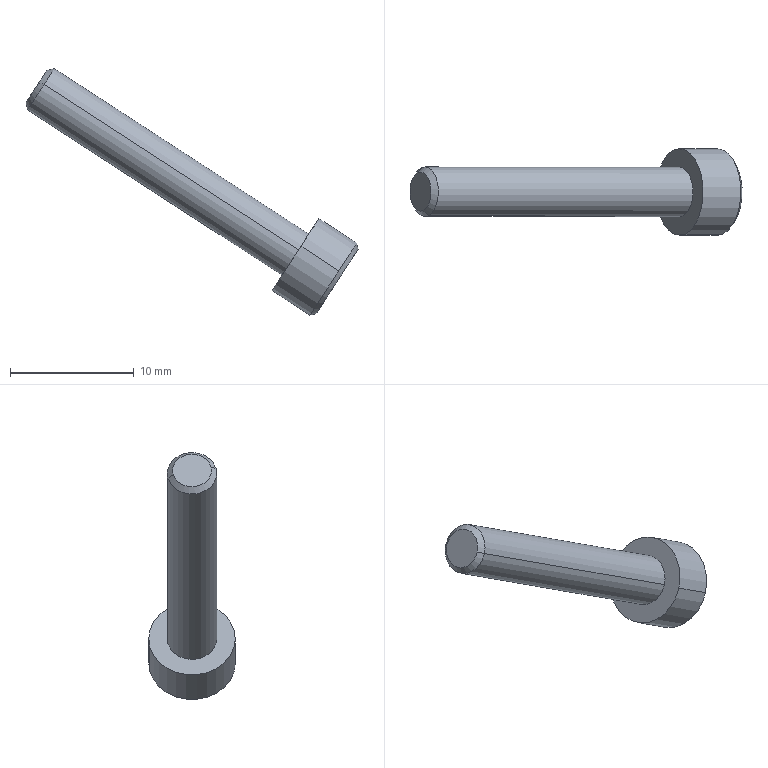Component | SolidWorks | ScrewTAC21-M4-L25(YIHEDA)-1 | 1 solid | 25 faces | box 26.89 x 7 x 19.98 mm | volume 448 mm3 | plane 15 | cone 6 | cylinder 4 | commonest cylinder face diameters 7 x2 4 x2
STEP:
#1=CARTESIAN_POINT('',(3.54,-0.8802,10.973));
#2=VERTEX_POINT('',#1);
#3=CARTESIAN_POINT('',(3.556,-1.,10.997));
#4=VERTEX_POINT('',#3);
#5=CARTESIAN_POINT('',(3.548,-0.9403,10.985));
#6=DIRECTION('',(-0.8387,0.,0.5446));
#7=DIRECTION('',(-0.1266,0.9726,-0.195));
#8=AXIS2_PLACEMENT_3D('',#5,#6,#7);
#9=CIRCLE('',#8,0.06183);
#10=EDGE_CURVE('',#2,#4,#9,.T.);
#11=ORIENTED_EDGE('',*,*,#10,.F.);
#12=CARTESIAN_POINT('',(3.552,-0.8637,10.961));
#13=VERTEX_POINT('',#12);
#14=CARTESIAN_POINT('',(3.552,-0.8637,10.961));
#15=DIRECTION('',(0.5035,0.6877,-0.523));
#16=VECTOR('',#15,39.37);
#17=LINE('',#14,#16);
#18=EDGE_CURVE('',#2,#13,#17,.T.);
#19=ORIENTED_EDGE('',*,*,#18,.T.);
#20=CARTESIAN_POINT('',(3.572,-1.017,10.991));
#21=VERTEX_POINT('',#20);
#22=CARTESIAN_POINT('',(3.562,-0.9403,10.976));
#23=DIRECTION('',(-0.8387,0.,0.5446));
#24=DIRECTION('',(-0.1266,0.9726,-0.195));
#25=AXIS2_PLACEMENT_3D('',#22,#23,#24);
#26=CIRCLE('',#25,0.07874);
#27=EDGE_CURVE('',#13,#21,#26,.T.);
#28=ORIENTED_EDGE('',*,*,#27,.T.);
#29=CARTESIAN_POINT('',(3.572,-1.017,10.991));
#30=DIRECTION('',(0.6826,-0.6877,-0.2473));
#31=VECTOR('',#30,39.37);
#32=LINE('',#29,#31);
#33=EDGE_CURVE('',#4,#21,#32,.T.);
#34=ORIENTED_EDGE('',*,*,#33,.F.);
#35=EDGE_LOOP('',(#11,#19,#28,#34));
#36=FACE_OUTER_BOUND('',#35,.T.);
#37=CARTESIAN_POINT('',(3.562,-0.9403,10.976));
#38=DIRECTION('',(0.8387,-0.,-0.5446));
#39=DIRECTION('',(0.1266,-0.9726,0.195));
#40=AXIS2_PLACEMENT_3D('',#37,#38,#39);
#41=CONICAL_SURFACE('',#40,0.07874,0.7854);
#42=ADVANCED_FACE('',(#36),#41,.T.);
#43=CARTESIAN_POINT('',(4.49,-0.8197,10.339));
#44=VERTEX_POINT('',#43);
#45=CARTESIAN_POINT('',(4.521,-1.061,10.388));
#46=VERTEX_POINT('',#45);
#47=CARTESIAN_POINT('',(4.506,-0.9403,10.363));
#48=DIRECTION('',(-0.8387,0.,0.5446));
#49=DIRECTION('',(-0.1266,0.9726,-0.195));
#50=AXIS2_PLACEMENT_3D('',#47,#48,#49);
#51=CIRCLE('',#50,0.124);
#52=EDGE_CURVE('',#44,#46,#51,.T.);
#53=ORIENTED_EDGE('',*,*,#52,.T.);
#54=CARTESIAN_POINT('',(4.512,-1.074,10.398));
#55=VERTEX_POINT('',#54);
#56=CARTESIAN_POINT('',(4.521,-1.061,10.388));
#57=DIRECTION('',(-0.5035,-0.6877,0.523));
#58=VECTOR('',#57,39.37);
#59=LINE('',#56,#58);
#60=EDGE_CURVE('',#46,#55,#59,.T.);
#61=ORIENTED_EDGE('',*,*,#60,.T.);
#62=CARTESIAN_POINT('',(4.477,-0.8063,10.344));
#63=VERTEX_POINT('',#62);
#64=CARTESIAN_POINT('',(4.494,-0.9403,10.371));
#65=DIRECTION('',(-0.8387,0.,0.5446));
#66=DIRECTION('',(-0.1266,0.9726,-0.195));
#67=AXIS2_PLACEMENT_3D('',#64,#65,#66);
#68=CIRCLE('',#67,0.1378);
#69=EDGE_CURVE('',#63,#55,#68,.T.);
#70=ORIENTED_EDGE('',*,*,#69,.F.);
#71=CARTESIAN_POINT('',(4.49,-0.8197,10.339));
#72=DIRECTION('',(-0.6826,0.6877,0.2473));
#73=VECTOR('',#72,39.37);
#74=LINE('',#71,#73);
#75=EDGE_CURVE('',#44,#63,#74,.T.);
#76=ORIENTED_EDGE('',*,*,#75,.F.);
#77=EDGE_LOOP('',(#53,#61,#70,#76));
#78=FACE_OUTER_BOUND('',#77,.T.);
#79=CARTESIAN_POINT('',(4.506,-0.9403,10.363));
#80=DIRECTION('',(-0.8387,0.,0.5446));
#81=DIRECTION('',(-0.1266,0.9726,-0.195));
#82=AXIS2_PLACEMENT_3D('',#79,#80,#81);
#83=CONICAL_SURFACE('',#82,0.124,0.7854);
#84=ADVANCED_FACE('',(#78),#83,.T.);
#85=CARTESIAN_POINT('',(4.391,-1.074,10.476));
#86=VERTEX_POINT('',#85);
#87=CARTESIAN_POINT('',(4.356,-0.8063,10.422));
#88=VERTEX_POINT('',#87);
#89=CARTESIAN_POINT('',(4.374,-0.9403,10.449));
#90=DIRECTION('',(-0.8387,0.,0.5446));
#91=DIRECTION('',(-0.1266,0.9726,-0.195));
#92=AXIS2_PLACEMENT_3D('',#89,#90,#91);
#93=CIRCLE('',#92,0.1378);
#94=EDGE_CURVE('',#86,#88,#93,.T.);
#95=ORIENTED_EDGE('',*,*,#94,.F.);
#96=CARTESIAN_POINT('',(4.391,-1.074,10.476));
#97=DIRECTION('',(0.8387,-0.,-0.5446));
#98=VECTOR('',#97,39.37);
#99=LINE('',#96,#98);
#100=EDGE_CURVE('',#86,#55,#99,.T.);
#101=ORIENTED_EDGE('',*,*,#100,.T.);
#102=CARTESIAN_POINT('',(4.494,-0.9403,10.371));
#103=DIRECTION('',(-0.8387,0.,0.5446));
#104=DIRECTION('',(-0.1266,0.9726,-0.195));
#105=AXIS2_PLACEMENT_3D('',#102,#103,#104);
#106=CIRCLE('',#105,0.1378);
#107=EDGE_CURVE('',#55,#63,#106,.T.);
#108=ORIENTED_EDGE('',*,*,#107,.T.);
#109=CARTESIAN_POINT('',(4.356,-0.8063,10.422));
#110=DIRECTION('',(0.8387,-0.,-0.5446));
#111=VECTOR('',#110,39.37);
#112=LINE('',#109,#111);
#113=EDGE_CURVE('',#88,#63,#112,.T.);
#114=ORIENTED_EDGE('',*,*,#113,.F.);
#115=EDGE_LOOP('',(#95,#101,#108,#114));
#116=FACE_OUTER_BOUND('',#115,.T.);
#117=CARTESIAN_POINT('',(4.374,-0.9403,10.449));
#118=DIRECTION('',(0.8387,-0.,-0.5446));
#119=DIRECTION('',(-0.1266,0.9726,-0.195));
#120=AXIS2_PLACEMENT_3D('',#117,#118,#119);
#121=CYLINDRICAL_SURFACE('',#120,0.1378);
#122=ADVANCED_FACE('',(#116),#121,.T.);
#123=CARTESIAN_POINT('',(4.411,-0.9403,10.425));
#124=VERTEX_POINT('',#123);
#125=CARTESIAN_POINT('',(4.471,-0.9266,10.454));
#126=VERTEX_POINT('',#125);
#127=CARTESIAN_POINT('',(4.471,-0.9266,10.454));
#128=DIRECTION('',(0.8781,0.2013,0.4341));
#129=VECTOR('',#128,39.37);
#130=LINE('',#127,#129);
#131=EDGE_CURVE('',#124,#126,#130,.T.);
#132=ORIENTED_EDGE('',*,*,#131,.F.);
#133=CARTESIAN_POINT('',(4.408,-0.954,10.358));
#134=VERTEX_POINT('',#133);
#135=CARTESIAN_POINT('',(4.408,-0.954,10.358));
#136=DIRECTION('',(-0.03941,-0.2013,-0.9787));
#137=VECTOR('',#136,39.37);
#138=LINE('',#135,#137);
#139=EDGE_CURVE('',#124,#134,#138,.T.);
#140=ORIENTED_EDGE('',*,*,#139,.T.);
#141=CARTESIAN_POINT('',(4.409,-0.9235,10.359));
#142=VERTEX_POINT('',#141);
#143=CARTESIAN_POINT('',(4.44,-0.9403,10.406));
#144=DIRECTION('',(-0.8387,0.,0.5446));
#145=DIRECTION('',(0.1266,-0.9726,0.195));
#146=AXIS2_PLACEMENT_3D('',#143,#144,#145);
#147=CIRCLE('',#146,0.05906);
#148=EDGE_CURVE('',#142,#134,#147,.T.);
#149=ORIENTED_EDGE('',*,*,#148,.F.);
#150=CARTESIAN_POINT('',(4.432,-0.8829,10.395));
#151=VERTEX_POINT('',#150);
#152=CARTESIAN_POINT('',(4.44,-0.9403,10.406));
#153=DIRECTION('',(-0.8387,0.,0.5446));
#154=DIRECTION('',(0.1266,-0.9726,0.195));
#155=AXIS2_PLACEMENT_3D('',#152,#153,#154);
#156=CIRCLE('',#155,0.05906);
#157=EDGE_CURVE('',#151,#142,#156,.T.);
#158=ORIENTED_EDGE('',*,*,#157,.F.);
#159=CARTESIAN_POINT('',(4.463,-0.8997,10.442));
#160=VERTEX_POINT('',#159);
#161=CARTESIAN_POINT('',(4.44,-0.9403,10.406));
#162=DIRECTION('',(-0.8387,0.,0.5446));
#163=DIRECTION('',(0.1266,-0.9726,0.195));
#164=AXIS2_PLACEMENT_3D('',#161,#162,#163);
#165=CIRCLE('',#164,0.05906);
#166=EDGE_CURVE('',#160,#151,#165,.T.);
#167=ORIENTED_EDGE('',*,*,#166,.F.);
#168=CARTESIAN_POINT('',(4.44,-0.9403,10.406));
#169=DIRECTION('',(-0.8387,0.,0.5446));
#170=DIRECTION('',(0.1266,-0.9726,0.195));
#171=AXIS2_PLACEMENT_3D('',#168,#169,#170);
#172=CIRCLE('',#171,0.05906);
#173=EDGE_CURVE('',#126,#160,#172,.T.);
#174=ORIENTED_EDGE('',*,*,#173,.F.);
#175=EDGE_LOOP('',(#132,#140,#149,#158,#167,#174));
#176=FACE_OUTER_BOUND('',#175,.T.);
#177=CARTESIAN_POINT('',(4.44,-0.9403,10.406));
#178=DIRECTION('',(0.8387,-0.,-0.5446));
#179=DIRECTION('',(0.5297,0.2325,0.8157));
#180=AXIS2_PLACEMENT_3D('',#177,#178,#179);
#181=CONICAL_SURFACE('',#180,0.05906,1.047);
#182=ADVANCED_FACE('',(#176),#181,.F.);
#183=CARTESIAN_POINT('',(3.562,-0.9403,10.976));
#184=DIRECTION('',(-0.8387,0.,0.5446));
#185=DIRECTION('',(-0.1266,0.9726,-0.195));
#186=AXIS2_PLACEMENT_3D('',#183,#184,#185);
#187=CIRCLE('',#186,0.07874);
#188=EDGE_CURVE('',#21,#13,#187,.T.);
#189=ORIENTED_EDGE('',*,*,#188,.F.);
#190=CARTESIAN_POINT('',(4.384,-1.017,10.465));
#191=VERTEX_POINT('',#190);
#192=CARTESIAN_POINT('',(3.558,-1.017,11.001));
#193=DIRECTION('',(0.8387,-0.,-0.5446));
#194=VECTOR('',#193,39.37);
#195=LINE('',#192,#194);
#196=EDGE_CURVE('',#21,#191,#195,.T.);
#197=ORIENTED_EDGE('',*,*,#196,.T.);
#198=CARTESIAN_POINT('',(4.364,-0.8637,10.434));
#199=VERTEX_POINT('',#198);
#200=CARTESIAN_POINT('',(4.374,-0.9403,10.449));
#201=DIRECTION('',(-0.8387,0.,0.5446));
#202=DIRECTION('',(-0.1266,0.9726,-0.195));
#203=AXIS2_PLACEMENT_3D('',#200,#201,#202);
#204=CIRCLE('',#203,0.07874);
#205=EDGE_CURVE('',#191,#199,#204,.T.);
#206=ORIENTED_EDGE('',*,*,#205,.T.);
#207=CARTESIAN_POINT('',(3.538,-0.8637,10.97));
#208=DIRECTION('',(0.8387,-0.,-0.5446));
#209=VECTOR('',#208,39.37);
#210=LINE('',#207,#209);
#211=EDGE_CURVE('',#13,#199,#210,.T.);
#212=ORIENTED_EDGE('',*,*,#211,.F.);
#213=EDGE_LOOP('',(#189,#197,#206,#212));
#214=FACE_OUTER_BOUND('',#213,.T.);
#215=CARTESIAN_POINT('',(3.548,-0.9403,10.985));
#216=DIRECTION('',(0.8387,-0.,-0.5446));
#217=DIRECTION('',(-0.1266,0.9726,-0.195));
#218=AXIS2_PLACEMENT_3D('',#215,#216,#217);
#219=CYLINDRICAL_SURFACE('',#218,0.07874);
#220=ADVANCED_FACE('',(#214),#219,.T.);
#221=CARTESIAN_POINT('',(4.476,-0.9245,10.462));
#222=VERTEX_POINT('',#221);
#223=CARTESIAN_POINT('',(4.471,-0.9571,10.454));
#224=VERTEX_POINT('',#223);
#225=CARTESIAN_POINT('',(4.476,-0.9245,10.462));
#226=DIRECTION('',(-0.1552,-0.9585,-0.239));
#227=VECTOR('',#226,39.37);
#228=LINE('',#225,#227);
#229=EDGE_CURVE('',#222,#224,#228,.T.);
#230=ORIENTED_EDGE('',*,*,#229,.T.);
#231=CARTESIAN_POINT('',(4.44,-0.9403,10.406));
#232=DIRECTION('',(-0.8387,0.,0.5446));
#233=DIRECTION('',(0.1266,-0.9726,0.195));
#234=AXIS2_PLACEMENT_3D('',#231,#232,#233);
#235=CIRCLE('',#234,0.05906);
#236=EDGE_CURVE('',#224,#126,#235,.T.);
#237=ORIENTED_EDGE('',*,*,#236,.T.);
#238=ORIENTED_EDGE('',*,*,#173,.T.);
#239=CARTESIAN_POINT('',(4.45,-0.875,10.423));
#240=DIRECTION('',(0.3745,-0.7261,0.5767));
#241=VECTOR('',#240,39.37);
#242=LINE('',#239,#241);
#243=EDGE_CURVE('',#160,#222,#242,.T.);
#244=ORIENTED_EDGE('',*,*,#243,.T.);
#245=EDGE_LOOP('',(#230,#237,#238,#244));
#246=FACE_OUTER_BOUND('',#245,.T.);
#247=CARTESIAN_POINT('',(4.44,-0.9403,10.406));
#248=DIRECTION('',(0.8387,-0.,-0.5446));
#249=DIRECTION('',(0.1266,-0.9726,0.195));
#250=AXIS2_PLACEMENT_3D('',#247,#248,#249);
#251=PLANE('',#250);
#252=ADVANCED_FACE('',(#246),#251,.T.);
#253=ORIENTED_EDGE('',*,*,#196,.F.);
#254=ORIENTED_EDGE('',*,*,#27,.F.);
#255=ORIENTED_EDGE('',*,*,#211,.T.);
#256=CARTESIAN_POINT('',(4.374,-0.9403,10.449));
#257=DIRECTION('',(-0.8387,0.,0.5446));
#258=DIRECTION('',(-0.1266,0.9726,-0.195));
#259=AXIS2_PLACEMENT_3D('',#256,#257,#258);
#260=CIRCLE('',#259,0.07874);
#261=EDGE_CURVE('',#199,#191,#260,.T.);
#262=ORIENTED_EDGE('',*,*,#261,.T.);
#263=EDGE_LOOP('',(#253,#254,#255,#262));
#264=FACE_OUTER_BOUND('',#263,.T.);
#265=CARTESIAN_POINT('',(3.548,-0.9403,10.985));
#266=DIRECTION('',(0.8387,-0.,-0.5446));
#267=DIRECTION('',(-0.1266,0.9726,-0.195));
#268=AXIS2_PLACEMENT_3D('',#265,#266,#267);
#269=CYLINDRICAL_SURFACE('',#268,0.07874);
#270=ADVANCED_FACE('',(#264),#269,.T.);
#271=ORIENTED_EDGE('',*,*,#139,.F.);
#272=ORIENTED_EDGE('',*,*,#131,.T.);
#273=ORIENTED_EDGE('',*,*,#236,.F.);
#274=CARTESIAN_POINT('',(4.447,-0.9978,10.418));
#275=VERTEX_POINT('',#274);
#276=CARTESIAN_POINT('',(4.44,-0.9403,10.406));
#277=DIRECTION('',(-0.8387,0.,0.5446));
#278=DIRECTION('',(0.1266,-0.9726,0.195));
#279=AXIS2_PLACEMENT_3D('',#276,#277,#278);
#280=CIRCLE('',#279,0.05906);
#281=EDGE_CURVE('',#275,#224,#280,.T.);
#282=ORIENTED_EDGE('',*,*,#281,.F.);
#283=CARTESIAN_POINT('',(4.416,-0.9809,10.37));
#284=VERTEX_POINT('',#283);
#285=CARTESIAN_POINT('',(4.44,-0.9403,10.406));
#286=DIRECTION('',(-0.8387,0.,0.5446));
#287=DIRECTION('',(0.1266,-0.9726,0.195));
#288=AXIS2_PLACEMENT_3D('',#285,#286,#287);
#289=CIRCLE('',#288,0.05906);
#290=EDGE_CURVE('',#284,#275,#289,.T.);
#291=ORIENTED_EDGE('',*,*,#290,.F.);
#292=CARTESIAN_POINT('',(4.44,-0.9403,10.406));
#293=DIRECTION('',(-0.8387,0.,0.5446));
#294=DIRECTION('',(0.1266,-0.9726,0.195));
#295=AXIS2_PLACEMENT_3D('',#292,#293,#294);
#296=CIRCLE('',#295,0.05906);
#297=EDGE_CURVE('',#134,#284,#296,.T.);
#298=ORIENTED_EDGE('',*,*,#297,.F.);
#299=EDGE_LOOP('',(#271,#272,#273,#282,#291,#298));
#300=FACE_OUTER_BOUND('',#299,.T.);
#301=CARTESIAN_POINT('',(4.44,-0.9403,10.406));
#302=DIRECTION('',(0.8387,-0.,-0.5446));
#303=DIRECTION('',(0.5297,0.2325,0.8157));
#304=AXIS2_PLACEMENT_3D('',#301,#302,#303);
#305=CONICAL_SURFACE('',#304,0.05906,1.047);
#306=ADVANCED_FACE('',(#300),#305,.F.);
#307=CARTESIAN_POINT('',(4.48,-0.8908,10.324));
#308=VERTEX_POINT('',#307);
#309=CARTESIAN_POINT('',(4.516,-0.875,10.38));
#310=VERTEX_POINT('',#309);
#311=CARTESIAN_POINT('',(4.48,-0.8908,10.324));
#312=DIRECTION('',(0.5297,0.2325,0.8157));
#313=VECTOR('',#312,39.37);
#314=LINE('',#311,#313);
#315=EDGE_CURVE('',#308,#310,#314,.T.);
#316=ORIENTED_EDGE('',*,*,#315,.T.);
#317=CARTESIAN_POINT('',(4.45,-0.875,10.423));
#318=VERTEX_POINT('',#317);
#319=CARTESIAN_POINT('',(4.45,-0.875,10.423));
#320=DIRECTION('',(0.8387,-0.,-0.5446));
#321=VECTOR('',#320,39.37);
#322=LINE('',#319,#321);
#323=EDGE_CURVE('',#318,#310,#322,.T.);
#324=ORIENTED_EDGE('',*,*,#323,.F.);
#325=CARTESIAN_POINT('',(4.414,-0.8908,10.367));
#326=DIRECTION('',(0.5297,0.2325,0.8157));
#327=VECTOR('',#326,39.37);
#328=LINE('',#325,#327);
#329=EDGE_CURVE('',#151,#318,#328,.T.);
#330=ORIENTED_EDGE('',*,*,#329,.F.);
#331=CARTESIAN_POINT('',(4.414,-0.8908,10.367));
#332=VERTEX_POINT('',#331);
#333=CARTESIAN_POINT('',(4.414,-0.8908,10.367));
#334=DIRECTION('',(0.5297,0.2325,0.8157));
#335=VECTOR('',#334,39.37);
#336=LINE('',#333,#335);
#337=EDGE_CURVE('',#332,#151,#336,.T.);
#338=ORIENTED_EDGE('',*,*,#337,.F.);
#339=CARTESIAN_POINT('',(4.414,-0.8908,10.367));
#340=DIRECTION('',(0.8387,-0.,-0.5446));
#341=VECTOR('',#340,39.37);
#342=LINE('',#339,#341);
#343=EDGE_CURVE('',#332,#308,#342,.T.);
#344=ORIENTED_EDGE('',*,*,#343,.T.);
#345=EDGE_LOOP('',(#316,#324,#330,#338,#344));
#346=FACE_OUTER_BOUND('',#345,.T.);
#347=CARTESIAN_POINT('',(4.414,-0.8908,10.367));
#348=DIRECTION('',(-0.1266,0.9726,-0.195));
#349=DIRECTION('',(0.8387,-0.,-0.5446));
#350=AXIS2_PLACEMENT_3D('',#347,#348,#349);
#351=PLANE('',#350);
#352=ADVANCED_FACE('',(#346),#351,.F.);
#353=CARTESIAN_POINT('',(4.495,-1.006,10.347));
#354=VERTEX_POINT('',#353);
#355=CARTESIAN_POINT('',(4.47,-0.9562,10.308));
#356=VERTEX_POINT('',#355);
#357=CARTESIAN_POINT('',(4.495,-1.006,10.347));
#358=DIRECTION('',(-0.3745,0.7261,-0.5767));
#359=VECTOR('',#358,39.37);
#360=LINE('',#357,#359);
#361=EDGE_CURVE('',#354,#356,#360,.T.);
#362=ORIENTED_EDGE('',*,*,#361,.T.);
#363=CARTESIAN_POINT('',(4.404,-0.9562,10.351));
#364=VERTEX_POINT('',#363);
#365=CARTESIAN_POINT('',(4.404,-0.9562,10.351));
#366=DIRECTION('',(0.8387,-0.,-0.5446));
#367=VECTOR('',#366,39.37);
#368=LINE('',#365,#367);
#369=EDGE_CURVE('',#364,#356,#368,.T.);
#370=ORIENTED_EDGE('',*,*,#369,.F.);
#371=CARTESIAN_POINT('',(4.429,-1.006,10.39));
#372=DIRECTION('',(-0.3745,0.7261,-0.5767));
#373=VECTOR('',#372,39.37);
#374=LINE('',#371,#373);
#375=EDGE_CURVE('',#284,#364,#374,.T.);
#376=ORIENTED_EDGE('',*,*,#375,.F.);
#377=CARTESIAN_POINT('',(4.429,-1.006,10.39));
#378=VERTEX_POINT('',#377);
#379=CARTESIAN_POINT('',(4.429,-1.006,10.39));
#380=DIRECTION('',(-0.3745,0.7261,-0.5767));
#381=VECTOR('',#380,39.37);
#382=LINE('',#379,#381);
#383=EDGE_CURVE('',#378,#284,#382,.T.);
#384=ORIENTED_EDGE('',*,*,#383,.F.);
#385=CARTESIAN_POINT('',(4.429,-1.006,10.39));
#386=DIRECTION('',(0.8387,-0.,-0.5446));
#387=VECTOR('',#386,39.37);
#388=LINE('',#385,#387);
#389=EDGE_CURVE('',#378,#354,#388,.T.);
#390=ORIENTED_EDGE('',*,*,#389,.T.);
#391=EDGE_LOOP('',(#362,#370,#376,#384,#390));
#392=FACE_OUTER_BOUND('',#391,.T.);
#393=CARTESIAN_POINT('',(4.429,-1.006,10.39));
#394=DIRECTION('',(-0.3954,-0.6876,-0.6089));
#395=DIRECTION('',(-0.8387,0.,0.5446));
#396=AXIS2_PLACEMENT_3D('',#393,#394,#395);
#397=PLANE('',#396);
#398=ADVANCED_FACE('',(#392),#397,.F.);
#399=ORIENTED_EDGE('',*,*,#383,.T.);
#400=ORIENTED_EDGE('',*,*,#290,.T.);
#401=CARTESIAN_POINT('',(4.465,-0.9898,10.446));
#402=DIRECTION('',(-0.5297,-0.2325,-0.8157));
#403=VECTOR('',#402,39.37);
#404=LINE('',#401,#403);
#405=EDGE_CURVE('',#275,#378,#404,.T.);
#406=ORIENTED_EDGE('',*,*,#405,.T.);
#407=EDGE_LOOP('',(#399,#400,#406));
#408=FACE_OUTER_BOUND('',#407,.T.);
#409=CARTESIAN_POINT('',(4.44,-0.9403,10.406));
#410=DIRECTION('',(0.8387,-0.,-0.5446));
#411=DIRECTION('',(0.1266,-0.9726,0.195));
#412=AXIS2_PLACEMENT_3D('',#409,#410,#411);
#413=PLANE('',#412);
#414=ADVANCED_FACE('',(#408),#413,.T.);
#415=CARTESIAN_POINT('',(4.374,-0.9403,10.449));
#416=DIRECTION('',(-0.8387,0.,0.5446));
#417=DIRECTION('',(-0.1266,0.9726,-0.195));
#418=AXIS2_PLACEMENT_3D('',#415,#416,#417);
#419=CIRCLE('',#418,0.1378);
#420=EDGE_CURVE('',#88,#86,#419,.T.);
#421=ORIENTED_EDGE('',*,*,#420,.T.);
#422=ORIENTED_EDGE('',*,*,#94,.T.);
#423=EDGE_LOOP('',(#421,#422));
#424=FACE_OUTER_BOUND('',#423,.T.);
#425=ORIENTED_EDGE('',*,*,#261,.F.);
#426=ORIENTED_EDGE('',*,*,#205,.F.);
#427=EDGE_LOOP('',(#425,#426));
#428=FACE_BOUND('',#427,.T.);
#429=CARTESIAN_POINT('',(4.301,-0.9723,10.337));
#430=DIRECTION('',(0.8387,-0.,-0.5446));
#431=DIRECTION('',(0.1266,-0.9726,0.195));
#432=AXIS2_PLACEMENT_3D('',#429,#430,#431);
#433=PLANE('',#432);
#434=ADVANCED_FACE('',(#424,#428),#433,.F.);
#435=ORIENTED_EDGE('',*,*,#52,.F.);
#436=CARTESIAN_POINT('',(4.506,-0.9403,10.363));
#437=DIRECTION('',(-0.8387,0.,0.5446));
#438=DIRECTION('',(-0.1266,0.9726,-0.195));
#439=AXIS2_PLACEMENT_3D('',#436,#437,#438);
#440=CIRCLE('',#439,0.124);
#441=EDGE_CURVE('',#46,#44,#440,.T.);
#442=ORIENTED_EDGE('',*,*,#441,.F.);
#443=EDGE_LOOP('',(#435,#442));
#444=FACE_OUTER_BOUND('',#443,.T.);
#445=CARTESIAN_POINT('',(4.542,-0.9245,10.419));
#446=VERTEX_POINT('',#445);
#447=CARTESIAN_POINT('',(4.531,-0.9898,10.403));
#448=VERTEX_POINT('',#447);
#449=CARTESIAN_POINT('',(4.542,-0.9245,10.419));
#450=DIRECTION('',(-0.1552,-0.9585,-0.239));
#451=VECTOR('',#450,39.37);
#452=LINE('',#449,#451);
#453=EDGE_CURVE('',#446,#448,#452,.T.);
#454=ORIENTED_EDGE('',*,*,#453,.F.);
#455=CARTESIAN_POINT('',(4.516,-0.875,10.38));
#456=DIRECTION('',(0.3745,-0.7261,0.5767));
#457=VECTOR('',#456,39.37);
#458=LINE('',#455,#457);
#459=EDGE_CURVE('',#310,#446,#458,.T.);
#460=ORIENTED_EDGE('',*,*,#459,.F.);
#461=ORIENTED_EDGE('',*,*,#315,.F.);
#462=CARTESIAN_POINT('',(4.47,-0.9562,10.308));
#463=DIRECTION('',(0.1552,0.9585,0.239));
#464=VECTOR('',#463,39.37);
#465=LINE('',#462,#464);
#466=EDGE_CURVE('',#356,#308,#465,.T.);
#467=ORIENTED_EDGE('',*,*,#466,.F.);
#468=ORIENTED_EDGE('',*,*,#361,.F.);
#469=CARTESIAN_POINT('',(4.531,-0.9898,10.403));
#470=DIRECTION('',(-0.5297,-0.2325,-0.8157));
#471=VECTOR('',#470,39.37);
#472=LINE('',#469,#471);
#473=EDGE_CURVE('',#448,#354,#472,.T.);
#474=ORIENTED_EDGE('',*,*,#473,.F.);
#475=EDGE_LOOP('',(#454,#460,#461,#467,#468,#474));
#476=FACE_BOUND('',#475,.T.);
#477=CARTESIAN_POINT('',(4.506,-0.9403,10.363));
#478=DIRECTION('',(-0.8387,0.,0.5446));
#479=DIRECTION('',(0.5297,0.2325,0.8157));
#480=AXIS2_PLACEMENT_3D('',#477,#478,#479);
#481=PLANE('',#480);
#482=ADVANCED_FACE('',(#444,#476),#481,.F.);
#483=CARTESIAN_POINT('',(3.548,-0.9403,10.985));
#484=DIRECTION('',(-0.8387,0.,0.5446));
#485=DIRECTION('',(-0.1266,0.9726,-0.195));
#486=AXIS2_PLACEMENT_3D('',#483,#484,#485);
#487=CIRCLE('',#486,0.06183);
#488=EDGE_CURVE('',#4,#2,#487,.T.);
#489=ORIENTED_EDGE('',*,*,#488,.T.);
#490=ORIENTED_EDGE('',*,*,#10,.T.);
#491=EDGE_LOOP('',(#489,#490));
#492=FACE_OUTER_BOUND('',#491,.T.);
#493=CARTESIAN_POINT('',(3.516,-0.9547,10.935));
#494=DIRECTION('',(0.8387,-0.,-0.5446));
#495=DIRECTION('',(0.1266,-0.9726,0.195));
#496=AXIS2_PLACEMENT_3D('',#493,#494,#495);
#497=PLANE('',#496);
#498=ADVANCED_FACE('',(#492),#497,.F.);
#499=ORIENTED_EDGE('',*,*,#100,.F.);
#500=ORIENTED_EDGE('',*,*,#420,.F.);
#501=ORIENTED_EDGE('',*,*,#113,.T.);
#502=ORIENTED_EDGE('',*,*,#69,.T.);
#503=EDGE_LOOP('',(#499,#500,#501,#502));
#504=FACE_OUTER_BOUND('',#503,.T.);
#505=CARTESIAN_POINT('',(4.374,-0.9403,10.449));
#506=DIRECTION('',(0.8387,-0.,-0.5446));
#507=DIRECTION('',(-0.1266,0.9726,-0.195));
#508=AXIS2_PLACEMENT_3D('',#505,#506,#507);
#509=CYLINDRICAL_SURFACE('',#508,0.1378);
#510=ADVANCED_FACE('',(#504),#509,.T.);
#511=ORIENTED_EDGE('',*,*,#459,.T.);
#512=CARTESIAN_POINT('',(4.476,-0.9245,10.462));
#513=DIRECTION('',(0.8387,-0.,-0.5446));
#514=VECTOR('',#513,39.37);
#515=LINE('',#512,#514);
#516=EDGE_CURVE('',#222,#446,#515,.T.);
#517=ORIENTED_EDGE('',*,*,#516,.F.);
#518=ORIENTED_EDGE('',*,*,#243,.F.);
#519=CARTESIAN_POINT('',(4.45,-0.875,10.423));
#520=DIRECTION('',(0.3745,-0.7261,0.5767));
#521=VECTOR('',#520,39.37);
#522=LINE('',#519,#521);
#523=EDGE_CURVE('',#318,#160,#522,.T.);
#524=ORIENTED_EDGE('',*,*,#523,.F.);
#525=ORIENTED_EDGE('',*,*,#323,.T.);
#526=EDGE_LOOP('',(#511,#517,#518,#524,#525));
#527=FACE_OUTER_BOUND('',#526,.T.);
#528=CARTESIAN_POINT('',(4.45,-0.875,10.423));
#529=DIRECTION('',(0.3954,0.6876,0.6089));
#530=DIRECTION('',(-0.3745,0.7261,-0.5767));
#531=AXIS2_PLACEMENT_3D('',#528,#529,#530);
#532=PLANE('',#531);
#533=ADVANCED_FACE('',(#527),#532,.F.);
#534=ORIENTED_EDGE('',*,*,#60,.F.);
#535=ORIENTED_EDGE('',*,*,#441,.T.);
#536=ORIENTED_EDGE('',*,*,#75,.T.);
#537=ORIENTED_EDGE('',*,*,#107,.F.);
#538=EDGE_LOOP('',(#534,#535,#536,#537));
#539=FACE_OUTER_BOUND('',#538,.T.);
#540=CARTESIAN_POINT('',(4.506,-0.9403,10.363));
#541=DIRECTION('',(-0.8387,0.,0.5446));
#542=DIRECTION('',(-0.1266,0.9726,-0.195));
#543=AXIS2_PLACEMENT_3D('',#540,#541,#542);
#544=CONICAL_SURFACE('',#543,0.124,0.7854);
#545=ADVANCED_FACE('',(#539),#544,.T.);
#546=ORIENTED_EDGE('',*,*,#453,.T.);
#547=CARTESIAN_POINT('',(4.465,-0.9898,10.446));
#548=VERTEX_POINT('',#547);
#549=CARTESIAN_POINT('',(4.465,-0.9898,10.446));
#550=DIRECTION('',(0.8387,-0.,-0.5446));
#551=VECTOR('',#550,39.37);
#552=LINE('',#549,#551);
#553=EDGE_CURVE('',#548,#448,#552,.T.);
#554=ORIENTED_EDGE('',*,*,#553,.F.);
#555=CARTESIAN_POINT('',(4.476,-0.9245,10.462));
#556=DIRECTION('',(-0.1552,-0.9585,-0.239));
#557=VECTOR('',#556,39.37);
#558=LINE('',#555,#557);
#559=EDGE_CURVE('',#224,#548,#558,.T.);
#560=ORIENTED_EDGE('',*,*,#559,.F.);
#561=ORIENTED_EDGE('',*,*,#229,.F.);
#562=ORIENTED_EDGE('',*,*,#516,.T.);
#563=EDGE_LOOP('',(#546,#554,#560,#561,#562));
#564=FACE_OUTER_BOUND('',#563,.T.);
#565=CARTESIAN_POINT('',(4.476,-0.9245,10.462));
#566=DIRECTION('',(0.5221,-0.285,0.8039));
#567=DIRECTION('',(-0.8387,0.,0.5446));
#568=AXIS2_PLACEMENT_3D('',#565,#566,#567);
#569=PLANE('',#568);
#570=ADVANCED_FACE('',(#564),#569,.F.);
#571=ORIENTED_EDGE('',*,*,#473,.T.);
#572=ORIENTED_EDGE('',*,*,#389,.F.);
#573=ORIENTED_EDGE('',*,*,#405,.F.);
#574=CARTESIAN_POINT('',(4.465,-0.9898,10.446));
#575=DIRECTION('',(-0.5297,-0.2325,-0.8157));
#576=VECTOR('',#575,39.37);
#577=LINE('',#574,#576);
#578=EDGE_CURVE('',#548,#275,#577,.T.);
#579=ORIENTED_EDGE('',*,*,#578,.F.);
#580=ORIENTED_EDGE('',*,*,#553,.T.);
#581=EDGE_LOOP('',(#571,#572,#573,#579,#580));
#582=FACE_OUTER_BOUND('',#581,.T.);
#583=CARTESIAN_POINT('',(4.465,-0.9898,10.446));
#584=DIRECTION('',(0.1266,-0.9726,0.195));
#585=DIRECTION('',(-0.5297,-0.2325,-0.8157));
#586=AXIS2_PLACEMENT_3D('',#583,#584,#585);
#587=PLANE('',#586);
#588=ADVANCED_FACE('',(#582),#587,.F.);
#589=ORIENTED_EDGE('',*,*,#578,.T.);
#590=ORIENTED_EDGE('',*,*,#281,.T.);
#591=ORIENTED_EDGE('',*,*,#559,.T.);
#592=EDGE_LOOP('',(#589,#590,#591));
#593=FACE_OUTER_BOUND('',#592,.T.);
#594=CARTESIAN_POINT('',(4.44,-0.9403,10.406));
#595=DIRECTION('',(0.8387,-0.,-0.5446));
#596=DIRECTION('',(0.1266,-0.9726,0.195));
#597=AXIS2_PLACEMENT_3D('',#594,#595,#596);
#598=PLANE('',#597);
#599=ADVANCED_FACE('',(#593),#598,.T.);
#600=ORIENTED_EDGE('',*,*,#523,.T.);
#601=ORIENTED_EDGE('',*,*,#166,.T.);
#602=ORIENTED_EDGE('',*,*,#329,.T.);
#603=EDGE_LOOP('',(#600,#601,#602));
#604=FACE_OUTER_BOUND('',#603,.T.);
#605=CARTESIAN_POINT('',(4.44,-0.9403,10.406));
#606=DIRECTION('',(0.8387,-0.,-0.5446));
#607=DIRECTION('',(0.1266,-0.9726,0.195));
#608=AXIS2_PLACEMENT_3D('',#605,#606,#607);
#609=PLANE('',#608);
#610=ADVANCED_FACE('',(#604),#609,.T.);
#611=ORIENTED_EDGE('',*,*,#337,.T.);
#612=ORIENTED_EDGE('',*,*,#157,.T.);
#613=CARTESIAN_POINT('',(4.404,-0.9562,10.351));
#614=DIRECTION('',(0.1552,0.9585,0.239));
#615=VECTOR('',#614,39.37);
#616=LINE('',#613,#615);
#617=EDGE_CURVE('',#142,#332,#616,.T.);
#618=ORIENTED_EDGE('',*,*,#617,.T.);
#619=EDGE_LOOP('',(#611,#612,#618));
#620=FACE_OUTER_BOUND('',#619,.T.);
#621=CARTESIAN_POINT('',(4.44,-0.9403,10.406));
#622=DIRECTION('',(0.8387,-0.,-0.5446));
#623=DIRECTION('',(0.1266,-0.9726,0.195));
#624=AXIS2_PLACEMENT_3D('',#621,#622,#623);
#625=PLANE('',#624);
#626=ADVANCED_FACE('',(#620),#625,.T.);
#627=ORIENTED_EDGE('',*,*,#466,.T.);
#628=ORIENTED_EDGE('',*,*,#343,.F.);
#629=ORIENTED_EDGE('',*,*,#617,.F.);
#630=CARTESIAN_POINT('',(4.404,-0.9562,10.351));
#631=DIRECTION('',(0.1552,0.9585,0.239));
#632=VECTOR('',#631,39.37);
#633=LINE('',#630,#632);
#634=EDGE_CURVE('',#364,#142,#633,.T.);
#635=ORIENTED_EDGE('',*,*,#634,.F.);
#636=ORIENTED_EDGE('',*,*,#369,.T.);
#637=EDGE_LOOP('',(#627,#628,#629,#635,#636));
#638=FACE_OUTER_BOUND('',#637,.T.);
#639=CARTESIAN_POINT('',(4.404,-0.9562,10.351));
#640=DIRECTION('',(-0.5221,0.285,-0.8039));
#641=DIRECTION('',(0.8387,-0.,-0.5446));
#642=AXIS2_PLACEMENT_3D('',#639,#640,#641);
#643=PLANE('',#642);
#644=ADVANCED_FACE('',(#638),#643,.F.);
#645=ORIENTED_EDGE('',*,*,#18,.F.);
#646=ORIENTED_EDGE('',*,*,#488,.F.);
#647=ORIENTED_EDGE('',*,*,#33,.T.);
#648=ORIENTED_EDGE('',*,*,#188,.T.);
#649=EDGE_LOOP('',(#645,#646,#647,#648));
#650=FACE_OUTER_BOUND('',#649,.T.);
#651=CARTESIAN_POINT('',(3.562,-0.9403,10.976));
#652=DIRECTION('',(0.8387,-0.,-0.5446));
#653=DIRECTION('',(0.1266,-0.9726,0.195));
#654=AXIS2_PLACEMENT_3D('',#651,#652,#653);
#655=CONICAL_SURFACE('',#654,0.07874,0.7854);
#656=ADVANCED_FACE('',(#650),#655,.T.);
#657=ORIENTED_EDGE('',*,*,#634,.T.);
#658=ORIENTED_EDGE('',*,*,#148,.T.);
#659=ORIENTED_EDGE('',*,*,#297,.T.);
#660=ORIENTED_EDGE('',*,*,#375,.T.);
#661=EDGE_LOOP('',(#657,#658,#659,#660));
#662=FACE_OUTER_BOUND('',#661,.T.);
#663=CARTESIAN_POINT('',(4.44,-0.9403,10.406));
#664=DIRECTION('',(0.8387,-0.,-0.5446));
#665=DIRECTION('',(0.1266,-0.9726,0.195));
#666=AXIS2_PLACEMENT_3D('',#663,#664,#665);
#667=PLANE('',#666);
#668=ADVANCED_FACE('',(#662),#667,.T.);
#669=CLOSED_SHELL('',(#42,#84,#122,#182,#220,#252,#270,#306,#352,#398,#414,#434,#482,#498,#510,#533,#545,#570,#588,#599,#610,#626,#644,#656,#668));
#670=MANIFOLD_SOLID_BREP('',#669);
#671=CARTESIAN_POINT('',(0.,0.,0.));
#672=DIRECTION('',(0.,0.,1.));
#673=DIRECTION('',(1.,0.,0.));
#674=AXIS2_PLACEMENT_3D('',#671,#672,#673);
#675=(LENGTH_UNIT()NAMED_UNIT(*)SI_UNIT($,.METRE.));
#676=LENGTH_MEASURE_WITH_UNIT(LENGTH_MEASURE(0.0254),#675);
#677=DIMENSIONAL_EXPONENTS(1.,0.,0.,0.,0.,0.,0.);
#678=(CONVERSION_BASED_UNIT('',#676)LENGTH_UNIT()NAMED_UNIT(#677));
#679=UNCERTAINTY_MEASURE_WITH_UNIT(LENGTH_MEASURE(0.00001),#678,'','');
#680=(NAMED_UNIT(*)PLANE_ANGLE_UNIT()SI_UNIT($,.RADIAN.));
#681=(NAMED_UNIT(*)SI_UNIT($,.STERADIAN.)SOLID_ANGLE_UNIT());
#682=(GEOMETRIC_REPRESENTATION_CONTEXT(3)GLOBAL_UNCERTAINTY_ASSIGNED_CONTEXT((#679))GLOBAL_UNIT_ASSIGNED_CONTEXT((#678,#680,#681))REPRESENTATION_CONTEXT('',''));
#683=ADVANCED_BREP_SHAPE_REPRESENTATION('',(#670,#674),#682);
#684=COLOUR_RGB('',0.7922,0.8196,0.9333);
#685=FILL_AREA_STYLE_COLOUR('',#684);
#686=FILL_AREA_STYLE('',(#685));
#687=SURFACE_STYLE_FILL_AREA(#686);
#688=SURFACE_SIDE_STYLE('',(#687));
#689=SURFACE_STYLE_USAGE(.BOTH.,#688);
#690=PRESENTATION_STYLE_ASSIGNMENT((#689));
#691=STYLED_ITEM('',(#690),#670);
#692=PRESENTATION_LAYER_ASSIGNMENT('','',(#691));
#693=(LENGTH_UNIT()NAMED_UNIT(*)SI_UNIT($,.METRE.));
#694=LENGTH_MEASURE_WITH_UNIT(LENGTH_MEASURE(0.0254),#693);
#695=DIMENSIONAL_EXPONENTS(1.,0.,0.,0.,0.,0.,0.);
#696=(CONVERSION_BASED_UNIT('',#694)LENGTH_UNIT()NAMED_UNIT(#695));
#697=UNCERTAINTY_MEASURE_WITH_UNIT(LENGTH_MEASURE(0.00001),#696,'','');
#698=(NAMED_UNIT(*)PLANE_ANGLE_UNIT()SI_UNIT($,.RADIAN.));
#699=(NAMED_UNIT(*)SI_UNIT($,.STERADIAN.)SOLID_ANGLE_UNIT());
#700=(GEOMETRIC_REPRESENTATION_CONTEXT(3)GLOBAL_UNCERTAINTY_ASSIGNED_CONTEXT((#697))GLOBAL_UNIT_ASSIGNED_CONTEXT((#696,#698,#699))REPRESENTATION_CONTEXT('',''));
#701=MECHANICAL_DESIGN_GEOMETRIC_PRESENTATION_REPRESENTATION('',(#691),#700);